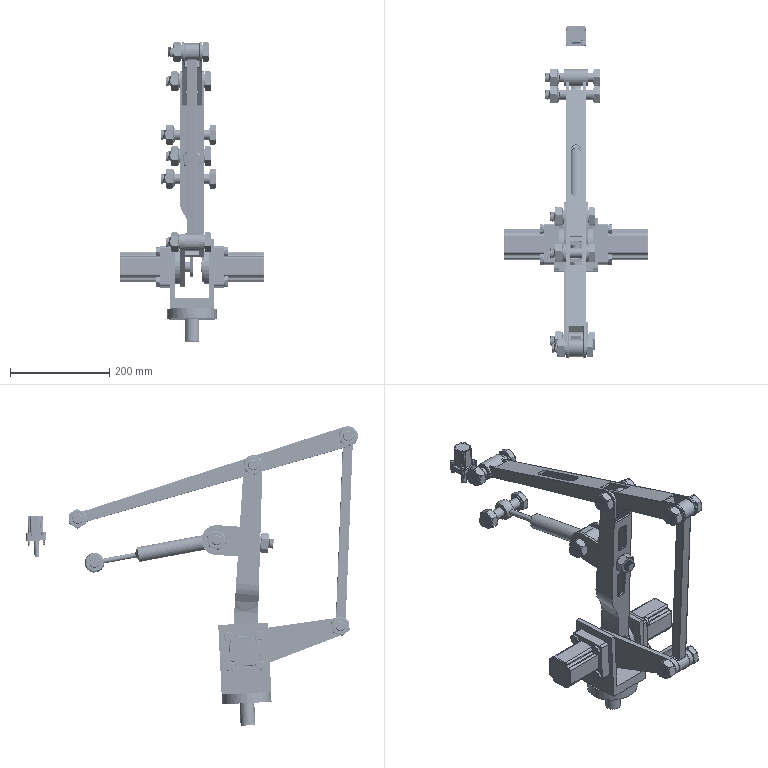Assembly | NX | mm | 66 component files | 85 solids | 1381 faces | box 290 x 668.74 x 603.36 mm | volume 2973642 mm3 | cylinder 587 | plane 553 | spline 121 | torus 86 | cone 20 | sphere 13 | other 1 | commonest cylinder face diameters 10 x136 20 x121 2 x100 5 x56 8 x36 4 x28 22 x16 17.5 x14
Bill of materials:
unnamed part 1 | 1 |  | Flanged block: square base flange with rounded corners and four corner through-holes, with a tall prismatic body rising from it. The body's cross-section is roughly square with stepped or notched corners, and the edges are rounded.
unnamed part 2 | 1 |  | Plain solid cylindrical rod with flat ends. One side view shows a small, shallow, rounded-end flat or slot near one end.
unnamed part 3 | 2 |  | Flanged rectangular body: square end flange with rounded corners, four corner through-holes, and a central round hole with a circular counterbore or recess on the flange face. A prismatic body with longitudinal edge grooves extends from the back of the flange.
unnamed part 4 | 2 |  | Hex-head bolt with a chamfered hexagonal head, a plain cylindrical shank, and threads on the end section only (partially threaded).
unnamed part 5 | 4 |  | Hex-head bolt with a chamfered hexagonal head, an unthreaded shank, and a threaded end section. One view looks along the axis from the thread end toward the head.
unnamed part 6 | 7 |  | Hexagonal nut with a central threaded through-hole and chamfered corners on both faces.
unnamed part 7 | 1 |  | Elongated arm or link: a forked (clevis-like) end with two parallel tines each carrying a hole, a web pierced by two rectangular slots and a central round hole, and a narrowing section ending in a single round eye boss with a hole.
unnamed part 8 | 1 |  | U-shaped clevis bracket: a flat base with two parallel side plates that have rounded (D-shaped) ends and coaxial through-holes, plus a hole through the base.
unnamed part 9 | 1 |  | Hex-head bolt, partially threaded, with a chamfered hexagonal head, a smooth shank, and a threaded end section.
unnamed part 10 | 1 |  | Yoke or fork bracket: two parallel rectangular side plates on a base, forming a U. Each plate has a central round hole and four smaller holes in a rectangular pattern, with circular raised rings or bosses on the inner faces. Below the base is a circular disc and a short cylindrical shaft stub on the axis.
unnamed part 11 | 4 |  | Hex-head bolt, partially threaded, with a chamfered hexagonal head, an unthreaded shank, and a threaded tip section.
unnamed part 12 | 1 |  | Straight slender connecting link: a rectangular-section bar with a cylindrical eye boss at each end, each eye with a through-hole, and the hole axes parallel.
unnamed part 13 | 1 |  | Long, narrow, flat link bar. One end splits into a fork with two parallel lugs that share a cross hole. The other end has a single cylindrical eye boss. Along the length there is a rectangular pocket with a cross hole and an elongated slot.
unnamed part 14 | 1 |  | Plain solid cylindrical rod with flat ends. One side view shows a small, shallow elongated recess near one end.
unnamed part 15 | 4 |  | Flat annular ring, similar to a washer, with a central round through-hole and flat parallel faces.
unnamed part 16 | 1 |  | Flat lever plate that tapers from one end to the other. The wide end is rounded and has a through-hole, with a raised boss on one face. The narrow end has a fork of two parallel lugs with coaxial holes.
unnamed part 17 | 8 |  | Flat annular ring, similar to a washer, with a central round hole. It is relatively thick compared with its diameter.
unnamed part 18 | 8 |  | Hex-head bolt. The shank is plain near the head and threaded toward the end, and the tip is chamfered.
unnamed part 19 | 1 |  | Slender rod with a rounded ring-shaped eye at one end, which has a through-hole. The other end has a short cylindrical collar or head of larger diameter.
unnamed part 20 | 1 |  | Pin with a flat head that is rounded on one side and squared on the other, with a transverse through-hole. The cylindrical shank ends in a chamfered tip.
unnamed part 21 | 14 |  | Thin flat ring with a large inner diameter relative to its outer diameter, giving a narrow radial wall.
unnamed part 22 | 1 |  | Solid cylindrical pin with flat ends. Near one end there is a small elongated recess with rounded ends, such as a slot or flat.
Mates:
1. concentric | CCJ-005 1 edge | CCJ-004 1 edge
2. concentric | CCJ-006 1 edge | CCJ-005 1 edge
3. concentric | CCJ-007 1 edge | CCJ-006 1 edge
4. parallel | CCJ-007 1 face | CCJ-004 1 face
5. touch align | CCJ-004 1 face | CCJ-007 1 face
6. concentric | CCJ-008 1 edge | CCJ-007 1 edge
7. fix | CCJ-008 1 component
8. concentric | CCJ-010 1 edge | CCJ-004 1 edge
9. touch align | CCJ-012 1 face | CCJ-011 1 face
10. concentric | CCJ-015 14 edge | CCJ-005 1 edge
11. concentric | CCJ-015 13 edge | CCJ-005 1 edge
12. concentric | CCJ-004 1 edge | CCJ-015 12 edge
13. concentric | CCJ-015 11 edge | CCJ-004 1 edge
14. concentric | CCJ-016 7 edge | CCJ-015 13 edge
15. concentric | CCJ-015 11 edge | CCJ-017 4 edge
16. concentric | CCJ-016 6 edge | CCJ-015 12 edge
17. concentric | CCJ-013 1 edge | CCJ-015 14 edge
18. concentric | CCJ-015 10 edge | CCJ-007 1 edge
19. concentric | CCJ-015 9 edge | CCJ-007 1 edge
20. concentric | CCJ-017 3 edge | CCJ-015 10 edge
21. concentric | CCJ-016 5 edge | CCJ-015 9 edge
22. concentric | CCJ-014 2 edge | CCJ-015 8 edge
23. concentric | CCJ-014 1 edge | CCJ-015 7 edge
24. concentric | CCJ-016 4 edge | CCJ-015 6 edge
25. concentric | CCJ-016 3 edge | CCJ-015 5 edge
26. concentric | CCJ-015 4 edge | CCJ-010 1 edge
27. concentric | CCJ-015 3 edge | CCJ-010 1 edge
28. concentric | CCJ-016 2 edge | CCJ-015 4 edge
29. concentric | CCJ-017 2 edge | CCJ-015 3 edge
30. concentric | CCJ-015 1 edge | CCJ-004 1 edge
31. concentric | CCJ-016 1 edge | CCJ-015 1 edge
32. concentric | CCJ-017 1 edge | CCJ-015 2 edge
33. concentric | CCJ-010 1 edge | CCJ-015 2 edge
34. concentric | CCJ-010 1 edge | CCJ-011 1 edge
35. concentric | CCJ-018 2 edge | CCJ-008 1 edge
36. concentric | CCJ-008 1 edge | CCJ-018 1 edge
37. parallel | CCJ-018 1 edge | CCJ-008 1 edge
38. concentric | CCJ-023 4 edge | CCJ-021 1 edge
39. concentric | CCJ-023 3 edge | CCJ-021 1 edge
40. concentric | CCJ-023 2 edge | CCJ-021 1 edge
41. concentric | CCJ-023 1 edge | CCJ-021 1 edge
42. concentric | CCJ-024 4 edge | CCJ-023 4 edge
43. concentric | CCJ-024 3 edge | CCJ-023 3 edge
44. concentric | CCJ-024 2 edge | CCJ-023 2 edge
45. concentric | CCJ-024 1 edge | CCJ-023 1 edge
46. parallel | CCJ-018 2 edge | CCJ-008 1 edge
47. concentric | CCJ-025 8 edge | CCJ-018 2 edge
48. concentric | CCJ-025 7 edge | CCJ-018 2 edge
49. concentric | CCJ-025 6 edge | CCJ-018 2 edge
50. concentric | CCJ-025 5 edge | CCJ-018 2 edge
51. concentric | CCJ-025 4 edge | CCJ-018 1 edge
52. concentric | CCJ-025 3 edge | CCJ-018 1 edge
53. concentric | CCJ-025 2 edge | CCJ-018 1 edge
54. concentric | CCJ-025 1 edge | CCJ-018 1 edge